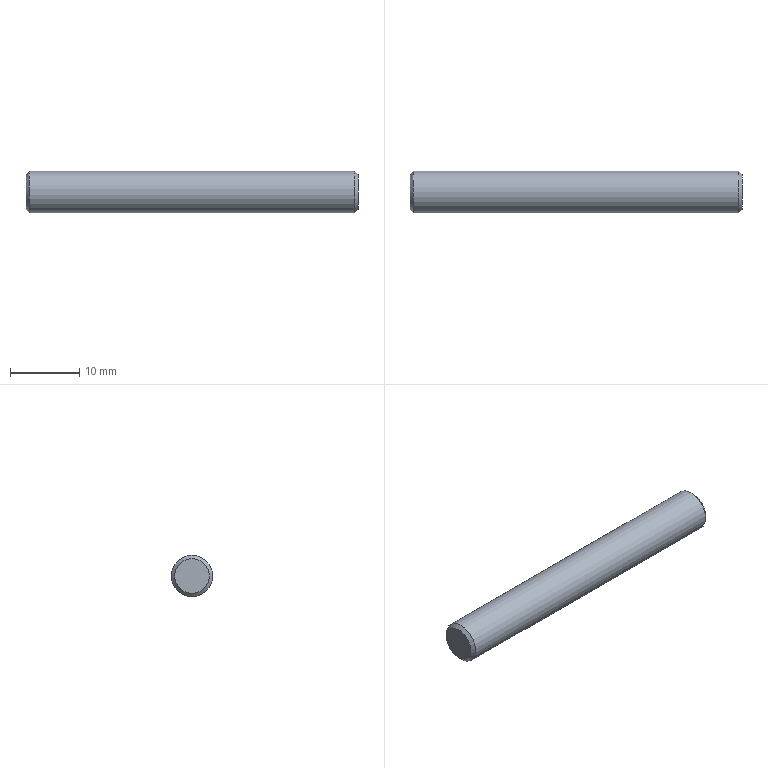Component | NX | HANDLE | 1 solid | 5 faces | box 48 x 6 x 6 mm | volume 1353 mm3 | plane 2 | cone 2 | cylinder 1 | commonest cylinder face diameters 6 x1
STEP:
#1=CARTESIAN_POINT('',(0.,0.,0.));
#2=DIRECTION('',(0.,0.,1.));
#3=DIRECTION('',(1.,0.,0.));
#4=AXIS2_PLACEMENT_3D('',#1,#2,#3);
#5=CARTESIAN_POINT('',(-31.505,167.895,146.614));
#6=VERTEX_POINT('',#5);
#7=CARTESIAN_POINT('',(-31.505,167.895,149.114));
#8=DIRECTION('',(-1.,0.,0.));
#9=DIRECTION('',(0.,0.,-1.));
#10=AXIS2_PLACEMENT_3D('',#7,#8,#9);
#11=CIRCLE('',#10,2.5);
#12=CARTESIAN_POINT('',(-31.505,167.895,149.114));
#13=DIRECTION('',(-1.,0.,0.));
#14=DIRECTION('',(0.,0.,-1.));
#15=AXIS2_PLACEMENT_3D('',#12,#13,#14);
#16=PLANE('',#15);
#17=CARTESIAN_POINT('',(0.,0.));
#18=DIRECTION('',(1.,0.));
#19=AXIS2_PLACEMENT_2D('',#17,#18);
#20=CIRCLE('',#19,2.5);
#21=(GEOMETRIC_REPRESENTATION_CONTEXT(2)PARAMETRIC_REPRESENTATION_CONTEXT()REPRESENTATION_CONTEXT('',''));
#22=DEFINITIONAL_REPRESENTATION('',(#20),#21);
#23=PCURVE('',#16,#22);
#24=CARTESIAN_POINT('',(-31.005,167.895,149.114));
#25=DIRECTION('',(1.,0.,0.));
#26=DIRECTION('',(0.,0.,1.));
#27=AXIS2_PLACEMENT_3D('',#24,#25,#26);
#28=CONICAL_SURFACE('',#27,3.,0.7854);
#29=CARTESIAN_POINT('',(9.425,-0.5));
#30=DIRECTION('',(-1.,0.));
#31=VECTOR('',#30,1.);
#32=LINE('',#29,#31);
#33=(GEOMETRIC_REPRESENTATION_CONTEXT(2)PARAMETRIC_REPRESENTATION_CONTEXT()REPRESENTATION_CONTEXT('',''));
#34=DEFINITIONAL_REPRESENTATION('',(#32),#33);
#35=PCURVE('',#28,#34);
#36=SURFACE_CURVE('',#11,(#23,#35),.PCURVE_S1.);
#37=EDGE_CURVE('',#6,#6,#36,.T.);
#38=ORIENTED_EDGE('',*,*,#37,.T.);
#39=EDGE_LOOP('',(#38));
#40=FACE_BOUND('',#39,.T.);
#41=ADVANCED_FACE('',(#40),#16,.T.);
#42=CARTESIAN_POINT('',(16.495,167.895,151.614));
#43=VERTEX_POINT('',#42);
#44=CARTESIAN_POINT('',(16.495,167.895,149.114));
#45=DIRECTION('',(1.,0.,0.));
#46=DIRECTION('',(0.,0.,1.));
#47=AXIS2_PLACEMENT_3D('',#44,#45,#46);
#48=CIRCLE('',#47,2.5);
#49=CARTESIAN_POINT('',(16.495,167.895,149.114));
#50=DIRECTION('',(1.,0.,0.));
#51=DIRECTION('',(0.,0.,1.));
#52=AXIS2_PLACEMENT_3D('',#49,#50,#51);
#53=PLANE('',#52);
#54=CARTESIAN_POINT('',(0.,0.));
#55=DIRECTION('',(1.,0.));
#56=AXIS2_PLACEMENT_2D('',#54,#55);
#57=CIRCLE('',#56,2.5);
#58=(GEOMETRIC_REPRESENTATION_CONTEXT(2)PARAMETRIC_REPRESENTATION_CONTEXT()REPRESENTATION_CONTEXT('',''));
#59=DEFINITIONAL_REPRESENTATION('',(#57),#58);
#60=PCURVE('',#53,#59);
#61=CARTESIAN_POINT('',(15.995,167.895,149.114));
#62=DIRECTION('',(-1.,0.,0.));
#63=DIRECTION('',(0.,0.,-1.));
#64=AXIS2_PLACEMENT_3D('',#61,#62,#63);
#65=CONICAL_SURFACE('',#64,3.,0.7854);
#66=CARTESIAN_POINT('',(9.425,-0.5));
#67=DIRECTION('',(-1.,0.));
#68=VECTOR('',#67,1.);
#69=LINE('',#66,#68);
#70=(GEOMETRIC_REPRESENTATION_CONTEXT(2)PARAMETRIC_REPRESENTATION_CONTEXT()REPRESENTATION_CONTEXT('',''));
#71=DEFINITIONAL_REPRESENTATION('',(#69),#70);
#72=PCURVE('',#65,#71);
#73=SURFACE_CURVE('',#48,(#60,#72),.PCURVE_S1.);
#74=EDGE_CURVE('',#43,#43,#73,.T.);
#75=ORIENTED_EDGE('',*,*,#74,.T.);
#76=EDGE_LOOP('',(#75));
#77=FACE_BOUND('',#76,.T.);
#78=ADVANCED_FACE('',(#77),#53,.T.);
#79=CARTESIAN_POINT('',(15.995,167.895,152.114));
#80=VERTEX_POINT('',#79);
#81=CARTESIAN_POINT('',(15.995,167.895,146.114));
#82=VERTEX_POINT('',#81);
#83=CARTESIAN_POINT('',(15.995,167.895,149.114));
#84=DIRECTION('',(-1.,0.,0.));
#85=DIRECTION('',(0.,0.,1.));
#86=AXIS2_PLACEMENT_3D('',#83,#84,#85);
#87=CIRCLE('',#86,3.);
#88=CARTESIAN_POINT('',(16.495,167.895,149.114));
#89=DIRECTION('',(-1.,0.,0.));
#90=DIRECTION('',(0.,0.,-1.));
#91=AXIS2_PLACEMENT_3D('',#88,#89,#90);
#92=CYLINDRICAL_SURFACE('',#91,3.);
#93=CARTESIAN_POINT('',(3.142,0.5));
#94=DIRECTION('',(1.,0.));
#95=VECTOR('',#94,1.);
#96=LINE('',#93,#95);
#97=(GEOMETRIC_REPRESENTATION_CONTEXT(2)PARAMETRIC_REPRESENTATION_CONTEXT()REPRESENTATION_CONTEXT('',''));
#98=DEFINITIONAL_REPRESENTATION('',(#96),#97);
#99=PCURVE('',#92,#98);
#100=CARTESIAN_POINT('',(3.142,0.));
#101=DIRECTION('',(1.,0.));
#102=VECTOR('',#101,1.);
#103=LINE('',#100,#102);
#104=(GEOMETRIC_REPRESENTATION_CONTEXT(2)PARAMETRIC_REPRESENTATION_CONTEXT()REPRESENTATION_CONTEXT('',''));
#105=DEFINITIONAL_REPRESENTATION('',(#103),#104);
#106=PCURVE('',#65,#105);
#107=SURFACE_CURVE('',#87,(#99,#106),.PCURVE_S1.);
#108=EDGE_CURVE('',#80,#82,#107,.T.);
#109=ORIENTED_EDGE('',*,*,#108,.T.);
#110=CARTESIAN_POINT('',(-31.005,167.895,146.114));
#111=VERTEX_POINT('',#110);
#112=CARTESIAN_POINT('',(15.995,167.895,146.114));
#113=CARTESIAN_POINT('',(-31.005,167.895,146.114));
#114=B_SPLINE_CURVE_WITH_KNOTS('',1,(#112,#113),.UNSPECIFIED.,.F.,.F.,(2,2),(0.5,47.5),.PIECEWISE_BEZIER_KNOTS.);
#115=CARTESIAN_POINT('',(6.283,0.));
#116=DIRECTION('',(0.,1.));
#117=VECTOR('',#116,1.);
#118=LINE('',#115,#117);
#119=(GEOMETRIC_REPRESENTATION_CONTEXT(2)PARAMETRIC_REPRESENTATION_CONTEXT()REPRESENTATION_CONTEXT('',''));
#120=DEFINITIONAL_REPRESENTATION('',(#118),#119);
#121=PCURVE('',#92,#120);
#122=CARTESIAN_POINT('',(0.,0.));
#123=DIRECTION('',(0.,1.));
#124=VECTOR('',#123,1.);
#125=LINE('',#122,#124);
#126=(GEOMETRIC_REPRESENTATION_CONTEXT(2)PARAMETRIC_REPRESENTATION_CONTEXT()REPRESENTATION_CONTEXT('',''));
#127=DEFINITIONAL_REPRESENTATION('',(#125),#126);
#128=PCURVE('',#92,#127);
#129=SEAM_CURVE('',#114,(#121,#128),.PCURVE_S1.);
#130=EDGE_CURVE('',#82,#111,#129,.T.);
#131=ORIENTED_EDGE('',*,*,#130,.T.);
#132=CARTESIAN_POINT('',(-31.005,167.895,149.114));
#133=DIRECTION('',(1.,0.,0.));
#134=DIRECTION('',(0.,0.,-1.));
#135=AXIS2_PLACEMENT_3D('',#132,#133,#134);
#136=CIRCLE('',#135,3.);
#137=CARTESIAN_POINT('',(6.283,47.5));
#138=DIRECTION('',(-1.,0.));
#139=VECTOR('',#138,1.);
#140=LINE('',#137,#139);
#141=(GEOMETRIC_REPRESENTATION_CONTEXT(2)PARAMETRIC_REPRESENTATION_CONTEXT()REPRESENTATION_CONTEXT('',''));
#142=DEFINITIONAL_REPRESENTATION('',(#140),#141);
#143=PCURVE('',#92,#142);
#144=CARTESIAN_POINT('',(3.142,0.));
#145=DIRECTION('',(1.,0.));
#146=VECTOR('',#145,1.);
#147=LINE('',#144,#146);
#148=(GEOMETRIC_REPRESENTATION_CONTEXT(2)PARAMETRIC_REPRESENTATION_CONTEXT()REPRESENTATION_CONTEXT('',''));
#149=DEFINITIONAL_REPRESENTATION('',(#147),#148);
#150=PCURVE('',#28,#149);
#151=SURFACE_CURVE('',#136,(#143,#150),.PCURVE_S1.);
#152=EDGE_CURVE('',#111,#111,#151,.T.);
#153=ORIENTED_EDGE('',*,*,#152,.T.);
#154=ORIENTED_EDGE('',*,*,#130,.F.);
#155=CARTESIAN_POINT('',(15.995,167.895,149.114));
#156=DIRECTION('',(-1.,0.,0.));
#157=DIRECTION('',(0.,0.,1.));
#158=AXIS2_PLACEMENT_3D('',#155,#156,#157);
#159=CIRCLE('',#158,3.);
#160=CARTESIAN_POINT('',(-3.142,0.5));
#161=DIRECTION('',(1.,0.));
#162=VECTOR('',#161,1.);
#163=LINE('',#160,#162);
#164=(GEOMETRIC_REPRESENTATION_CONTEXT(2)PARAMETRIC_REPRESENTATION_CONTEXT()REPRESENTATION_CONTEXT('',''));
#165=DEFINITIONAL_REPRESENTATION('',(#163),#164);
#166=PCURVE('',#92,#165);
#167=CARTESIAN_POINT('',(3.142,0.));
#168=DIRECTION('',(1.,0.));
#169=VECTOR('',#168,1.);
#170=LINE('',#167,#169);
#171=(GEOMETRIC_REPRESENTATION_CONTEXT(2)PARAMETRIC_REPRESENTATION_CONTEXT()REPRESENTATION_CONTEXT('',''));
#172=DEFINITIONAL_REPRESENTATION('',(#170),#171);
#173=PCURVE('',#65,#172);
#174=SURFACE_CURVE('',#159,(#166,#173),.PCURVE_S1.);
#175=EDGE_CURVE('',#82,#80,#174,.T.);
#176=ORIENTED_EDGE('',*,*,#175,.T.);
#177=EDGE_LOOP('',(#109,#131,#153,#154,#176));
#178=FACE_BOUND('',#177,.T.);
#179=ADVANCED_FACE('',(#178),#92,.T.);
#180=ORIENTED_EDGE('',*,*,#74,.F.);
#181=CARTESIAN_POINT('',(16.495,167.895,151.614));
#182=CARTESIAN_POINT('',(15.995,167.895,152.114));
#183=B_SPLINE_CURVE_WITH_KNOTS('',1,(#181,#182),.UNSPECIFIED.,.F.,.F.,(2,2),(-0.7071,0.),.PIECEWISE_BEZIER_KNOTS.);
#184=CARTESIAN_POINT('',(9.425,0.));
#185=DIRECTION('',(0.,1.));
#186=VECTOR('',#185,1.);
#187=LINE('',#184,#186);
#188=(GEOMETRIC_REPRESENTATION_CONTEXT(2)PARAMETRIC_REPRESENTATION_CONTEXT()REPRESENTATION_CONTEXT('',''));
#189=DEFINITIONAL_REPRESENTATION('',(#187),#188);
#190=PCURVE('',#65,#189);
#191=CARTESIAN_POINT('',(3.142,0.));
#192=DIRECTION('',(0.,1.));
#193=VECTOR('',#192,1.);
#194=LINE('',#191,#193);
#195=(GEOMETRIC_REPRESENTATION_CONTEXT(2)PARAMETRIC_REPRESENTATION_CONTEXT()REPRESENTATION_CONTEXT('',''));
#196=DEFINITIONAL_REPRESENTATION('',(#194),#195);
#197=PCURVE('',#65,#196);
#198=SEAM_CURVE('',#183,(#190,#197),.PCURVE_S1.);
#199=EDGE_CURVE('',#43,#80,#198,.T.);
#200=ORIENTED_EDGE('',*,*,#199,.T.);
#201=ORIENTED_EDGE('',*,*,#175,.F.);
#202=ORIENTED_EDGE('',*,*,#108,.F.);
#203=ORIENTED_EDGE('',*,*,#199,.F.);
#204=EDGE_LOOP('',(#180,#200,#201,#202,#203));
#205=FACE_BOUND('',#204,.T.);
#206=ADVANCED_FACE('',(#205),#65,.T.);
#207=ORIENTED_EDGE('',*,*,#37,.F.);
#208=CARTESIAN_POINT('',(-31.505,167.895,146.614));
#209=CARTESIAN_POINT('',(-31.005,167.895,146.114));
#210=B_SPLINE_CURVE_WITH_KNOTS('',1,(#208,#209),.UNSPECIFIED.,.F.,.F.,(2,2),(-0.7071,0.),.PIECEWISE_BEZIER_KNOTS.);
#211=CARTESIAN_POINT('',(9.425,0.));
#212=DIRECTION('',(0.,1.));
#213=VECTOR('',#212,1.);
#214=LINE('',#211,#213);
#215=(GEOMETRIC_REPRESENTATION_CONTEXT(2)PARAMETRIC_REPRESENTATION_CONTEXT()REPRESENTATION_CONTEXT('',''));
#216=DEFINITIONAL_REPRESENTATION('',(#214),#215);
#217=PCURVE('',#28,#216);
#218=CARTESIAN_POINT('',(3.142,0.));
#219=DIRECTION('',(0.,1.));
#220=VECTOR('',#219,1.);
#221=LINE('',#218,#220);
#222=(GEOMETRIC_REPRESENTATION_CONTEXT(2)PARAMETRIC_REPRESENTATION_CONTEXT()REPRESENTATION_CONTEXT('',''));
#223=DEFINITIONAL_REPRESENTATION('',(#221),#222);
#224=PCURVE('',#28,#223);
#225=SEAM_CURVE('',#210,(#217,#224),.PCURVE_S1.);
#226=EDGE_CURVE('',#6,#111,#225,.T.);
#227=ORIENTED_EDGE('',*,*,#226,.T.);
#228=ORIENTED_EDGE('',*,*,#152,.F.);
#229=ORIENTED_EDGE('',*,*,#226,.F.);
#230=EDGE_LOOP('',(#207,#227,#228,#229));
#231=FACE_BOUND('',#230,.T.);
#232=ADVANCED_FACE('',(#231),#28,.T.);
#233=CLOSED_SHELL('',(#41,#78,#179,#206,#232));
#234=MANIFOLD_SOLID_BREP('',#233);
#235=(LENGTH_UNIT()NAMED_UNIT(*)SI_UNIT(.MILLI.,.METRE.));
#236=UNCERTAINTY_MEASURE_WITH_UNIT(LENGTH_MEASURE(0.00001),#235,'','');
#237=(NAMED_UNIT(*)PLANE_ANGLE_UNIT()SI_UNIT($,.RADIAN.));
#238=(NAMED_UNIT(*)SI_UNIT($,.STERADIAN.)SOLID_ANGLE_UNIT());
#239=(GEOMETRIC_REPRESENTATION_CONTEXT(3)GLOBAL_UNCERTAINTY_ASSIGNED_CONTEXT((#236))GLOBAL_UNIT_ASSIGNED_CONTEXT((#235,#237,#238))REPRESENTATION_CONTEXT('',''));
#240=ADVANCED_BREP_SHAPE_REPRESENTATION('',(#4,#234),#239);